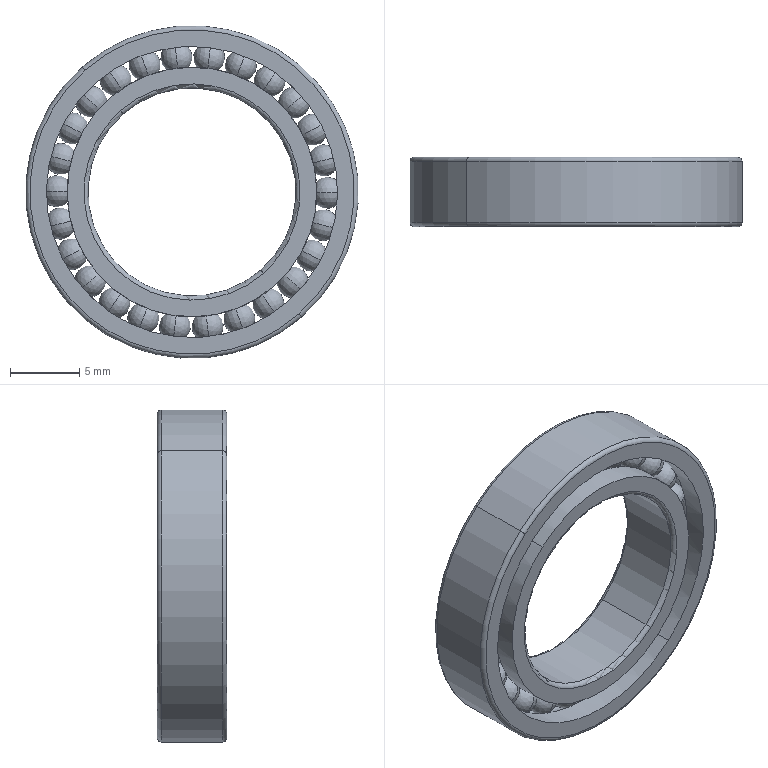Component | SolidWorks | CrankshaftOne-1_deep groove ball bearings gb-2 | 1 solid | 157 faces | volume 1018 mm3 | torus 89 | sphere 52 | cylinder 12 | plane 4 | commonest cylinder face diameters 21 x4 18 x4 24 x2 15 x2